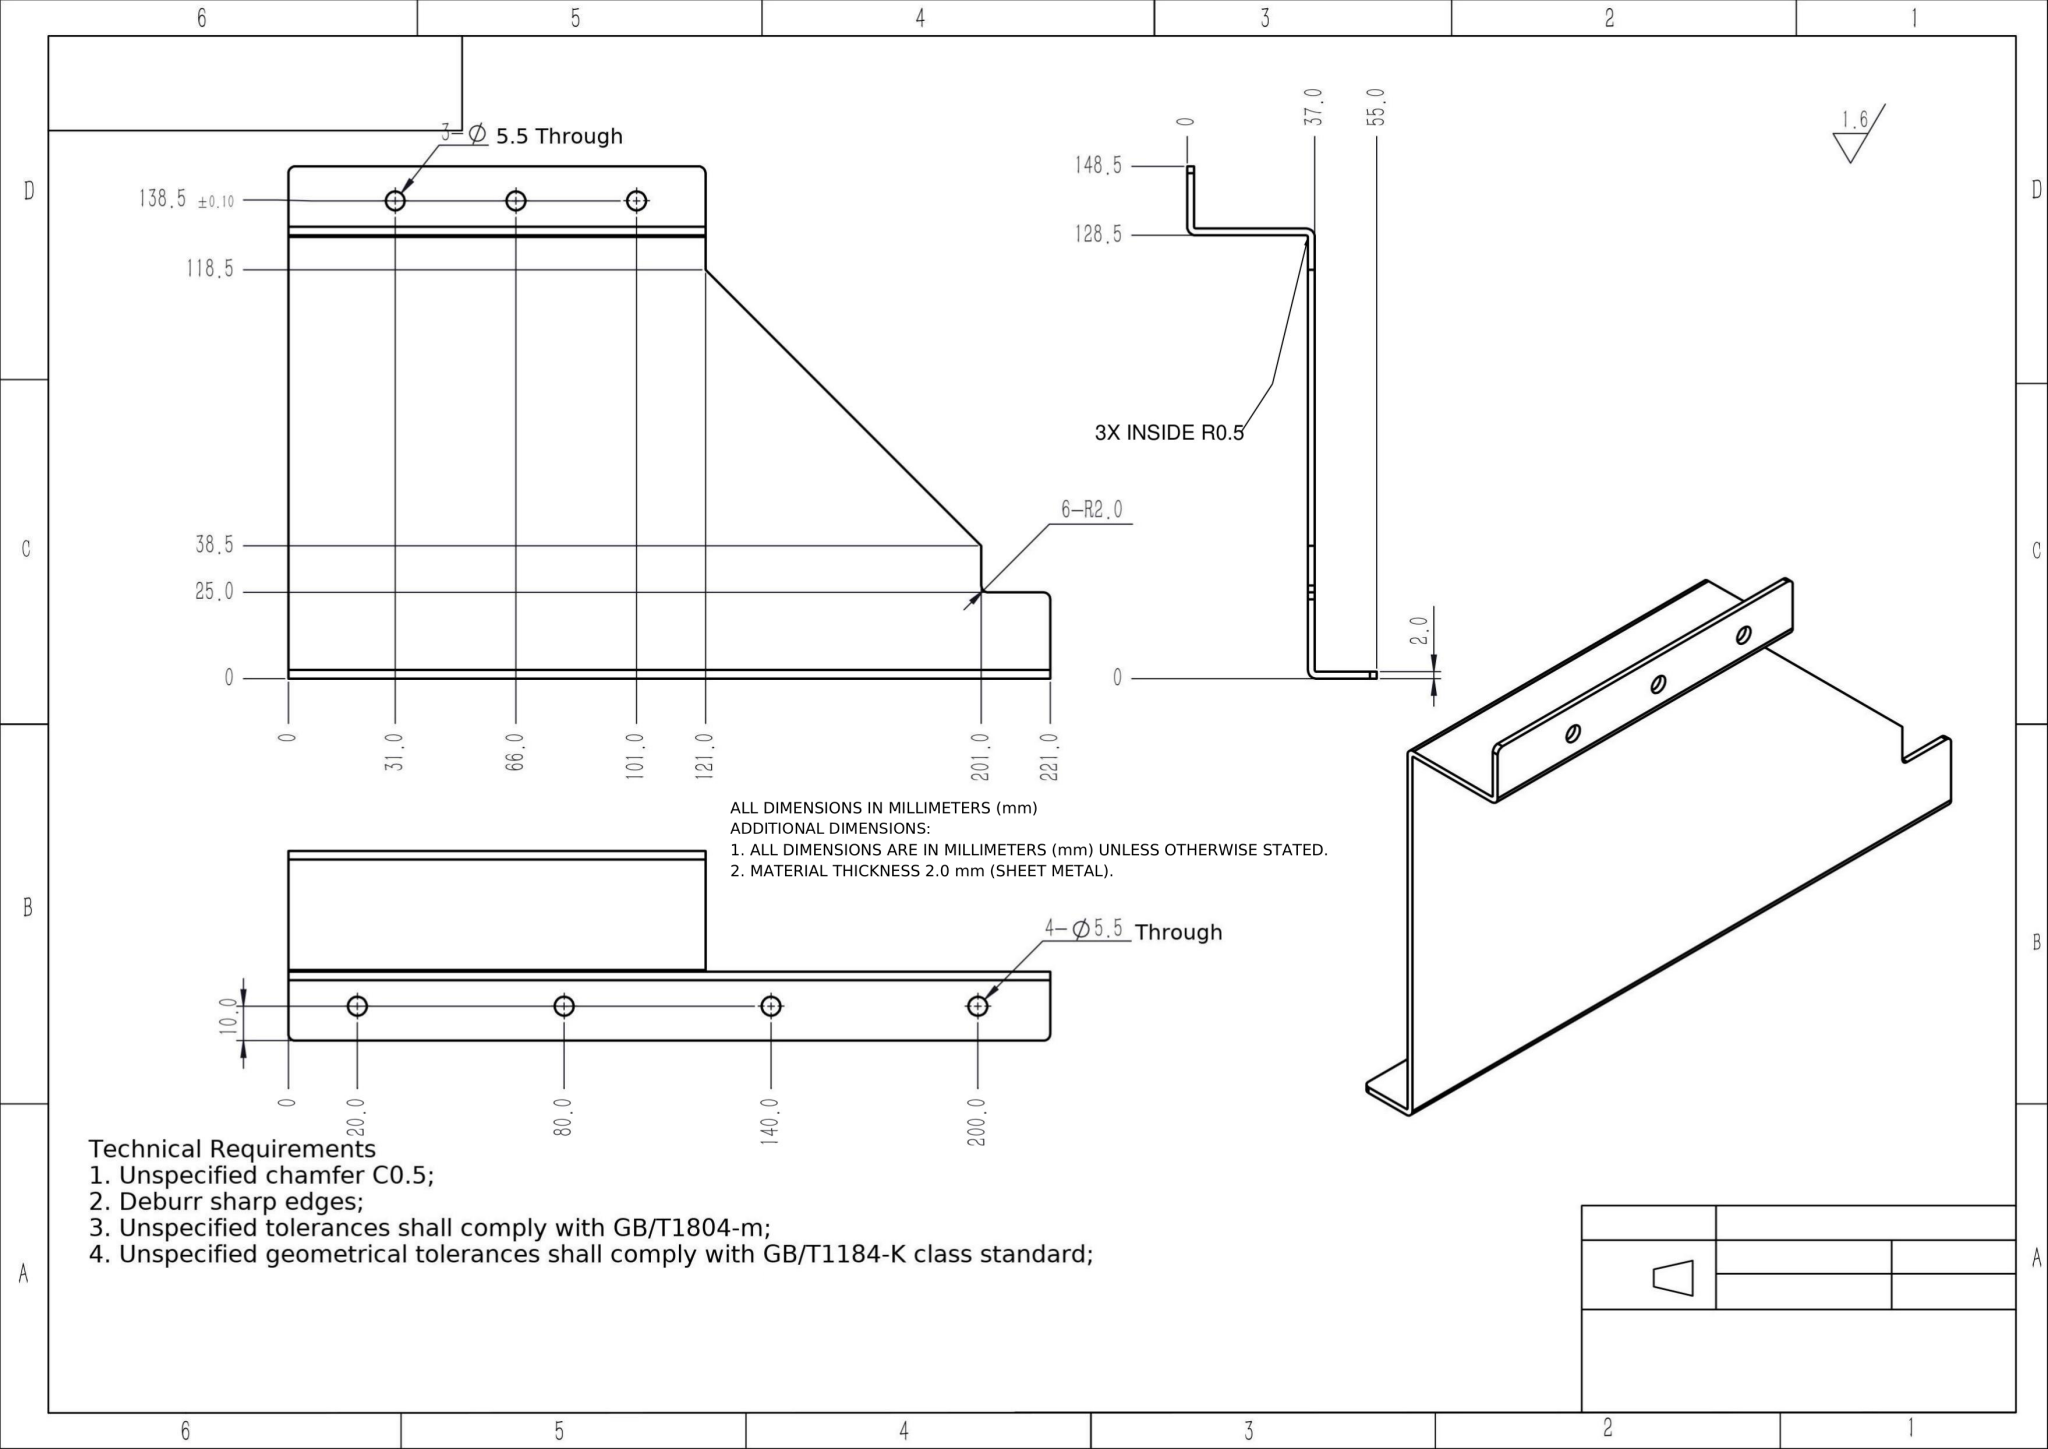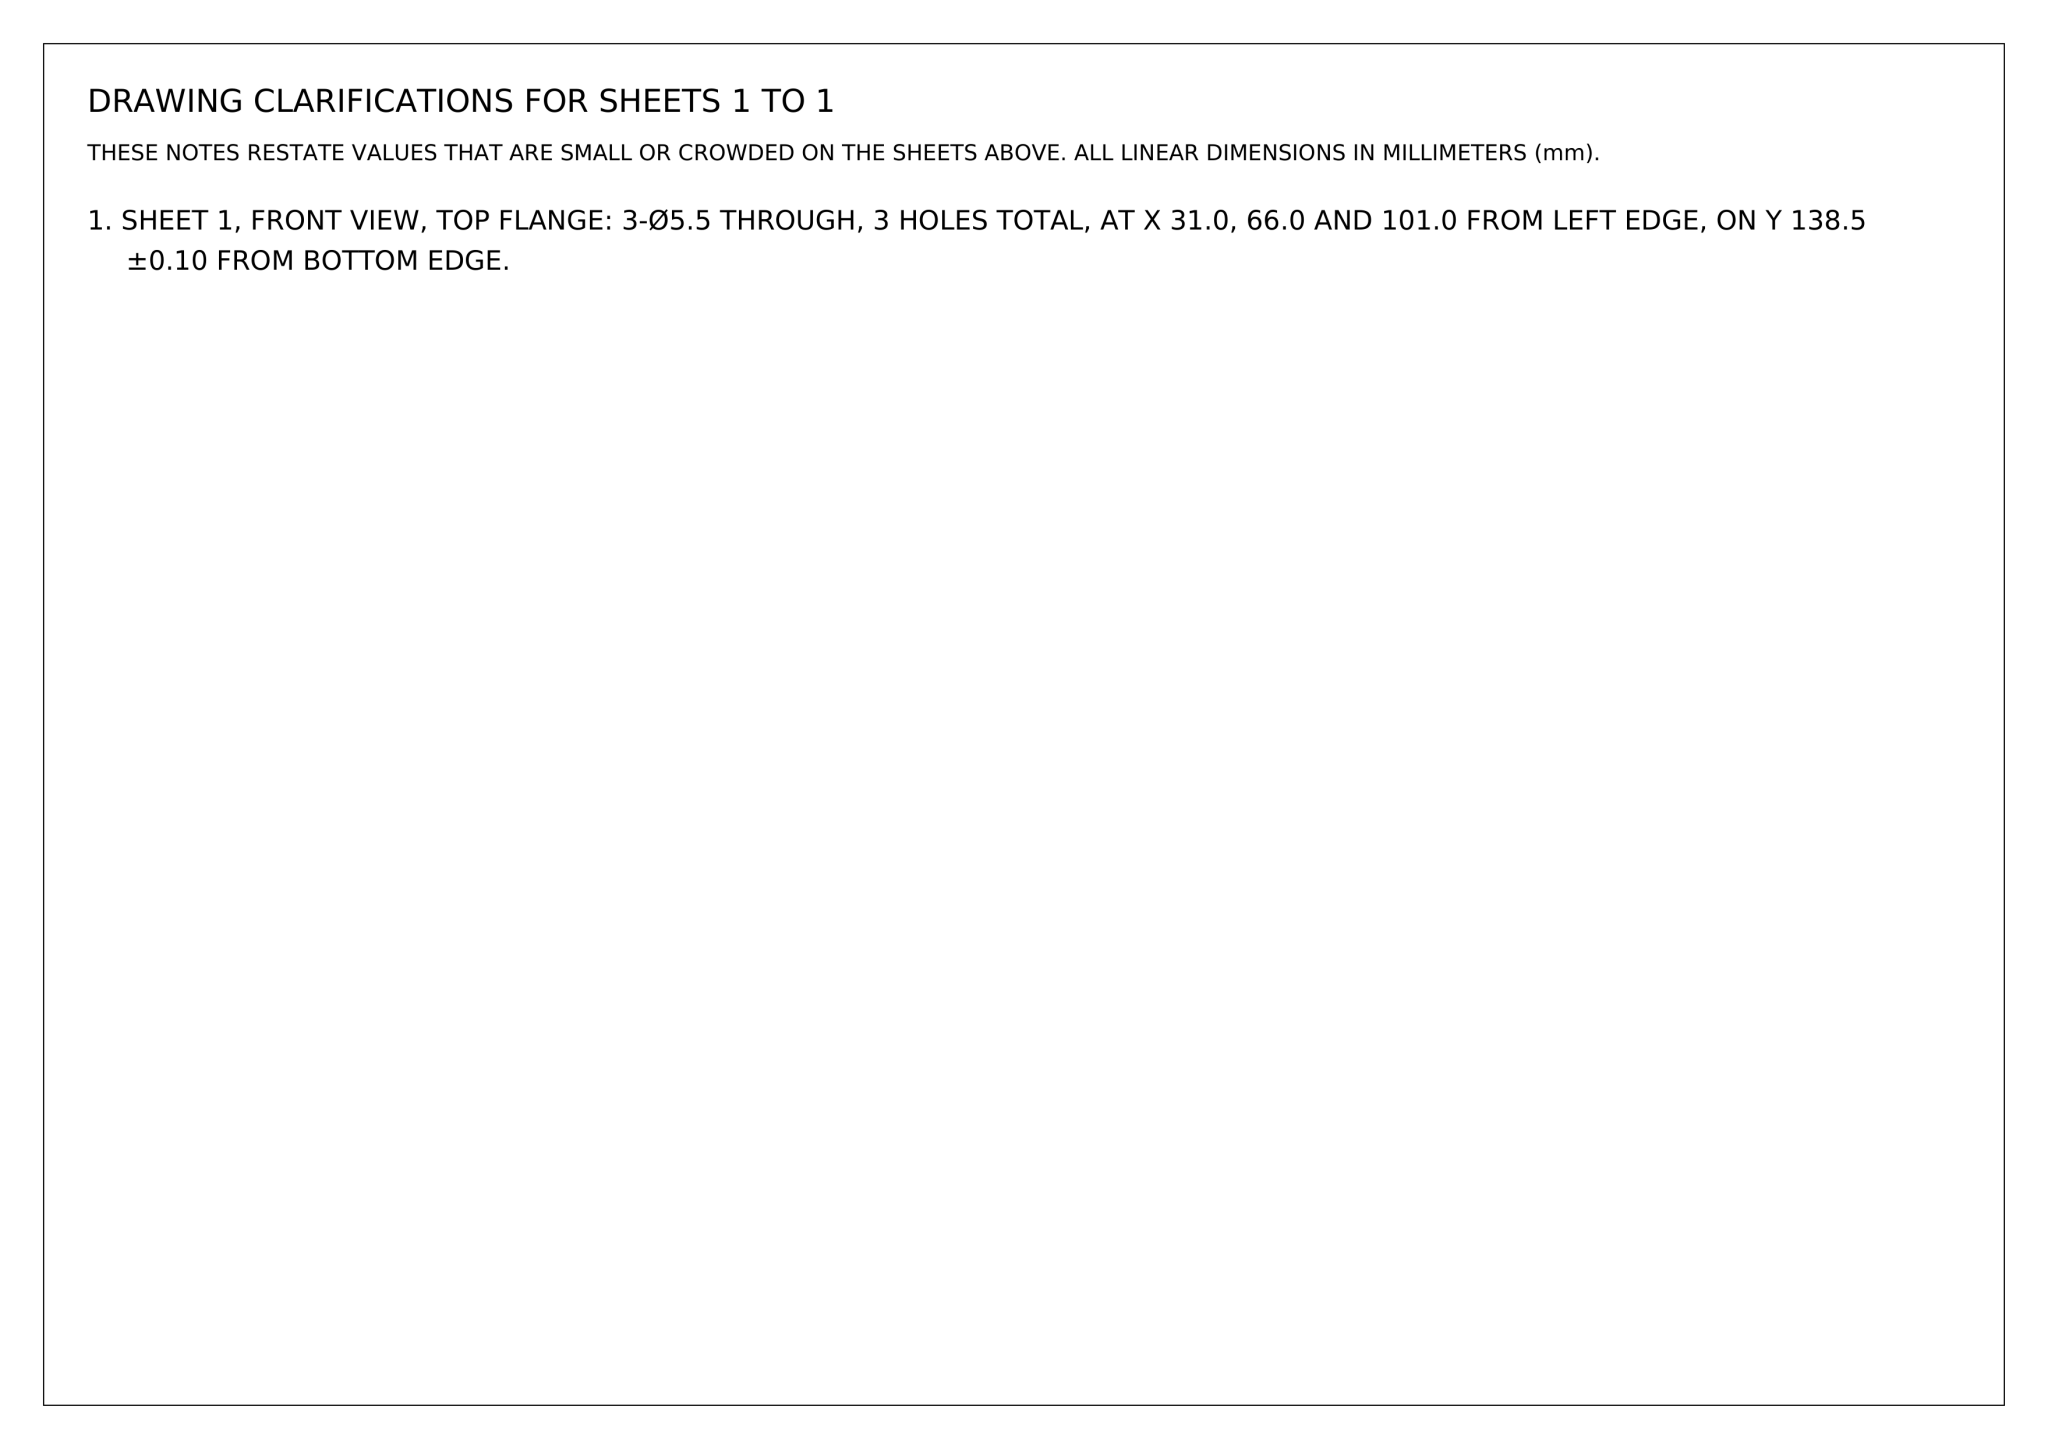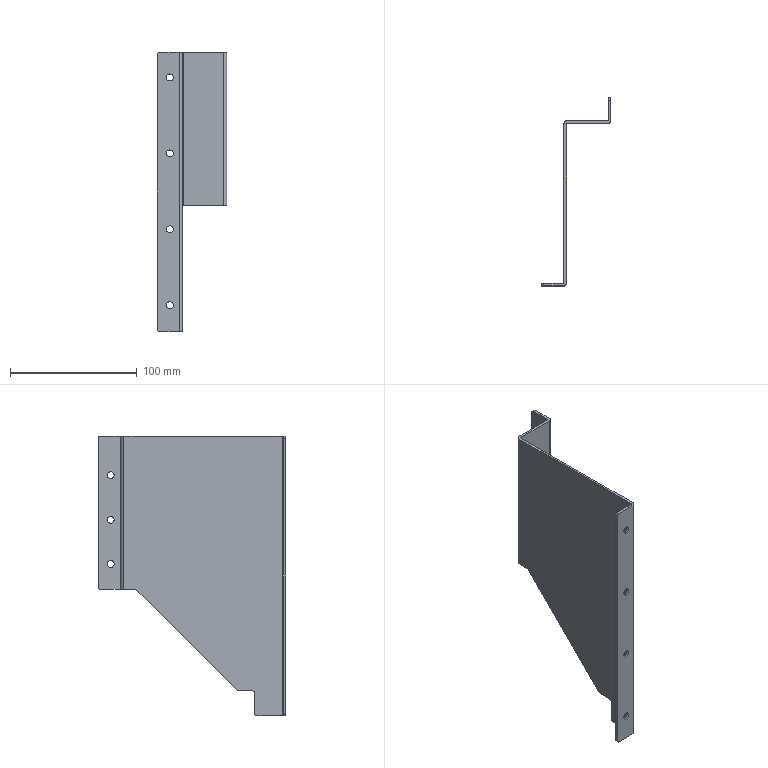Part | NX | mm | Gusseted U-Channel Wall Bracket | 1 solid | 42 faces | box 55 x 148.5 x 221 mm | volume 64987 mm3 | cylinder 26 | plane 16 | commonest cylinder face diameters 5.5 x14 4 x6 1 x3 5 x3